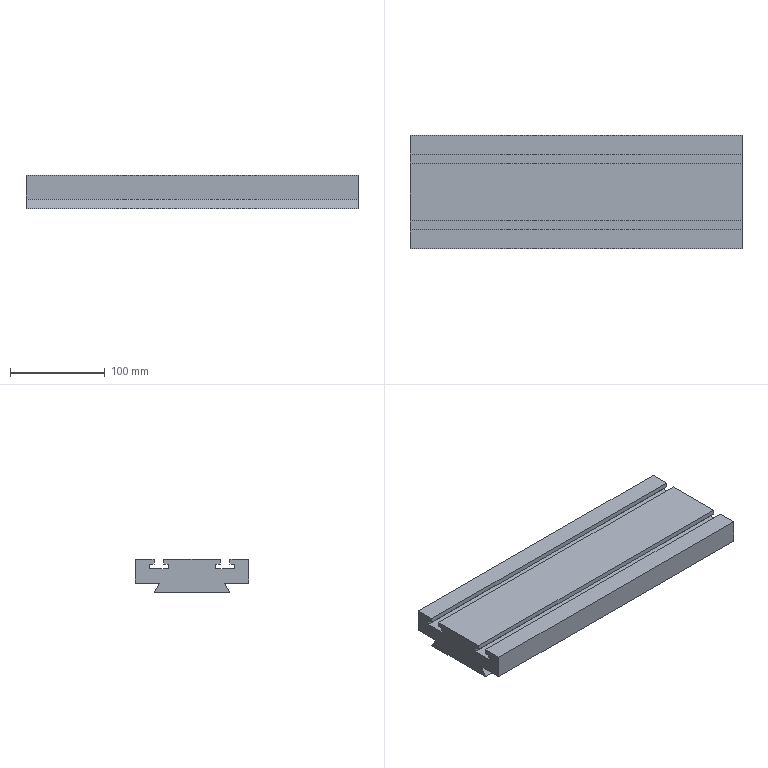Component | NX | WORK_TABLE | 1 solid | 40 faces | volume 833491 mm3 | plane 31 | cylinder 7 | cone 2 | commonest cylinder face diameters 20 x4 4.2 x2 18 x1